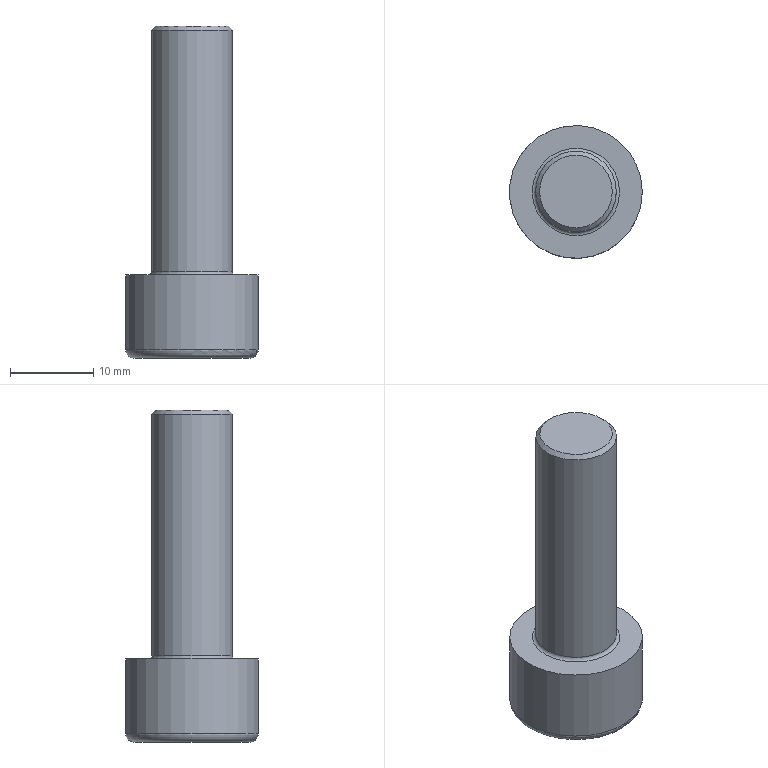Component | NX | SCREW_M10X30 | 1 solid | 27 faces | volume 3856 mm3 | plane 15 | cone 8 | cylinder 2 | torus 2 | commonest cylinder face diameters 9.732 x1 16 x1